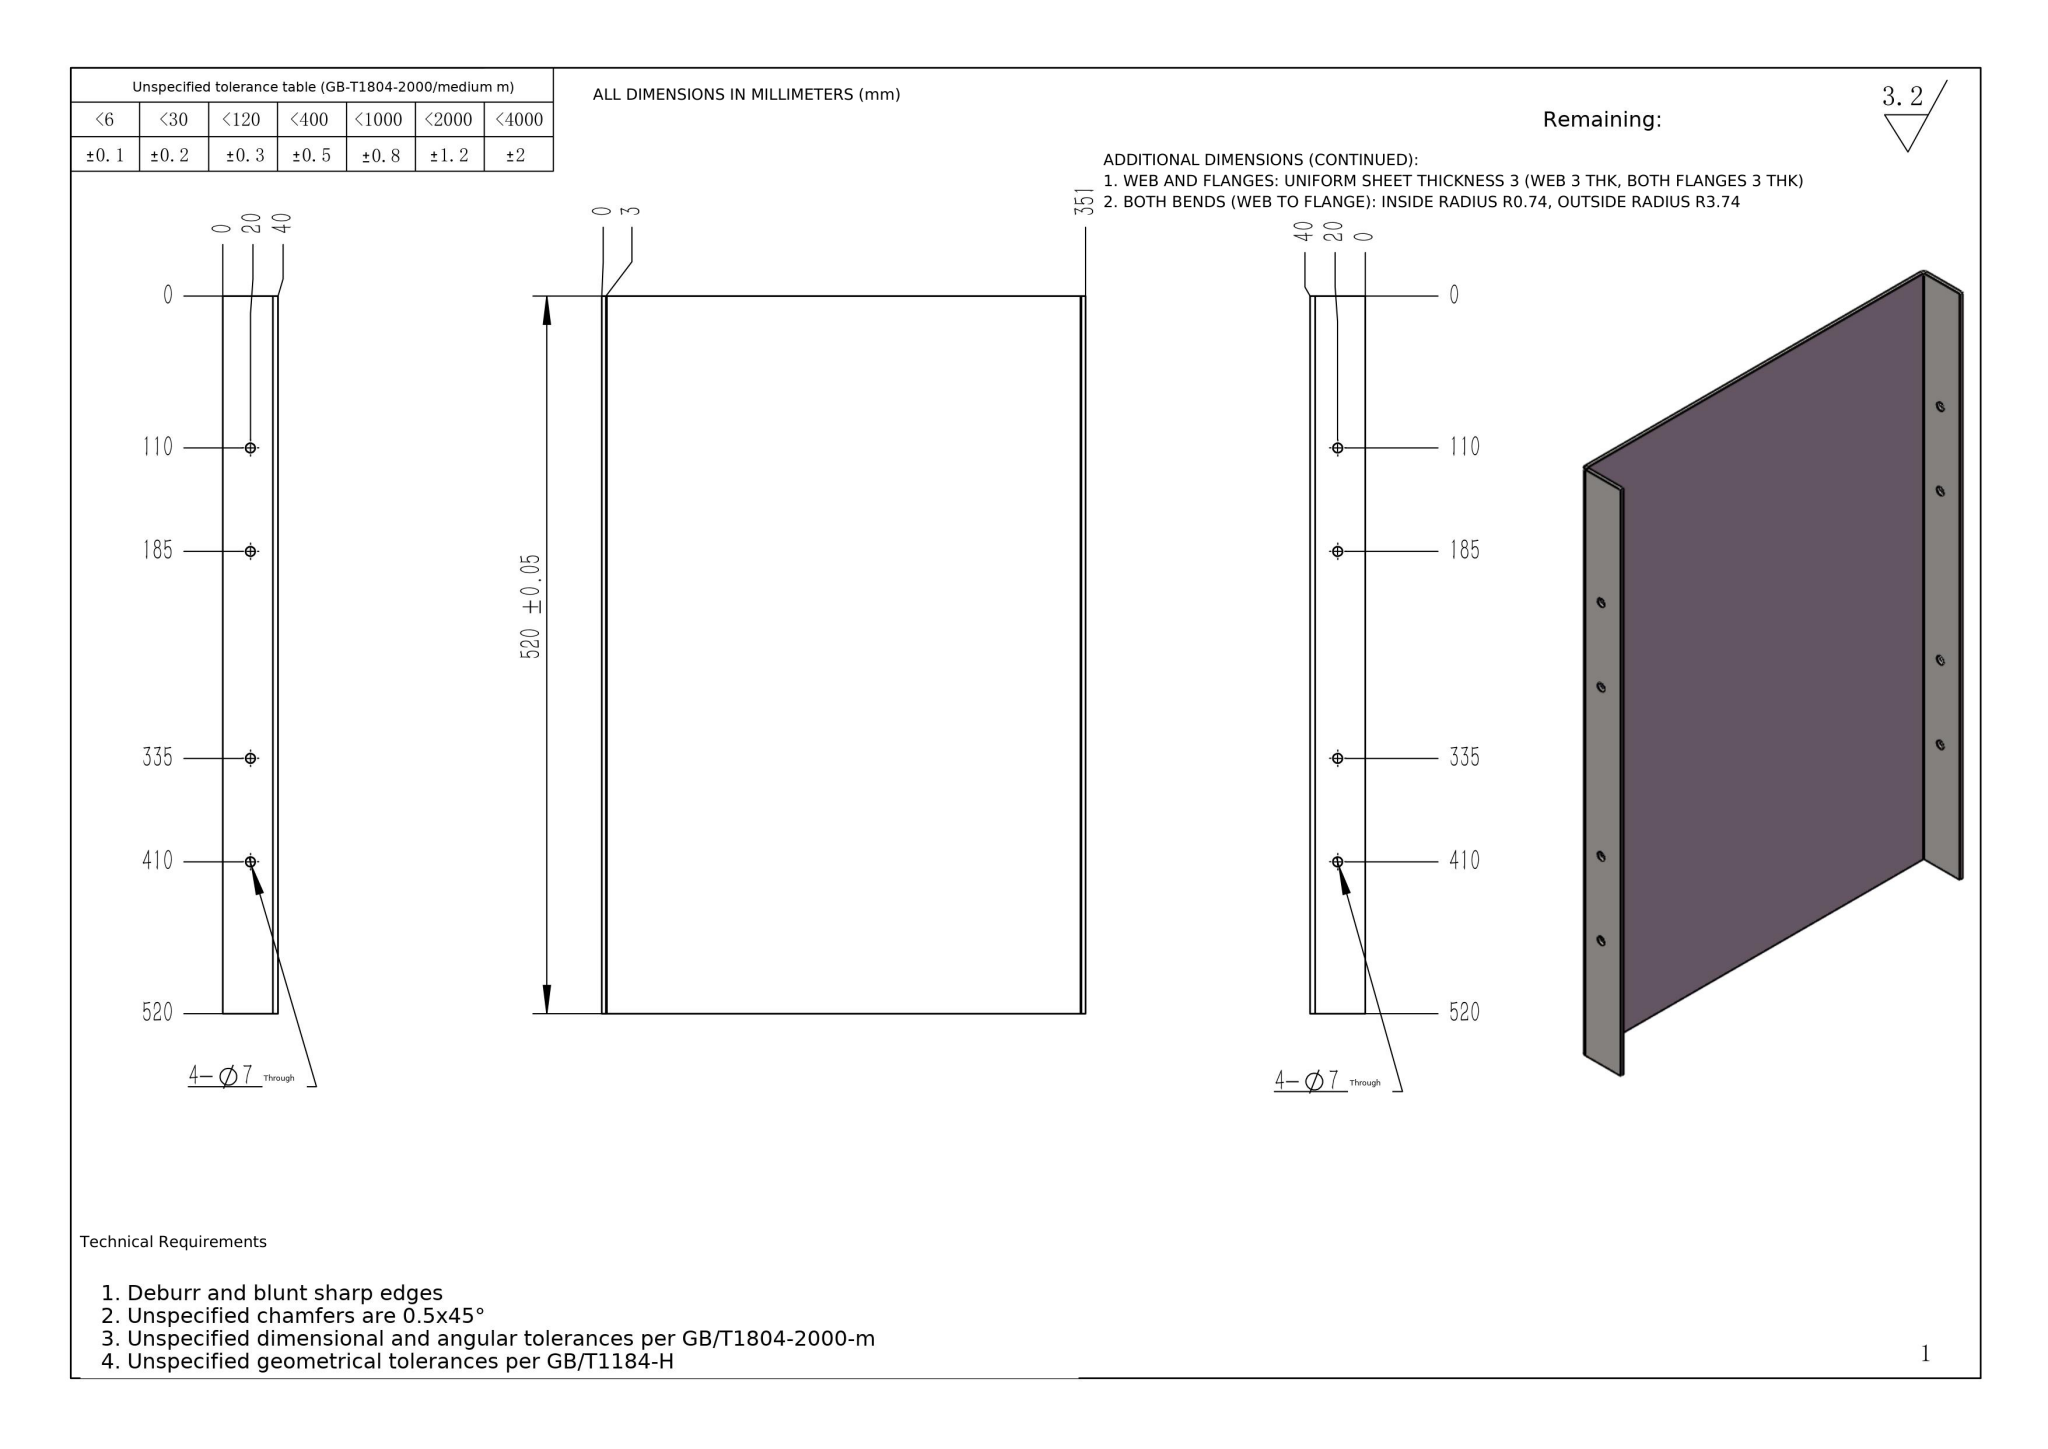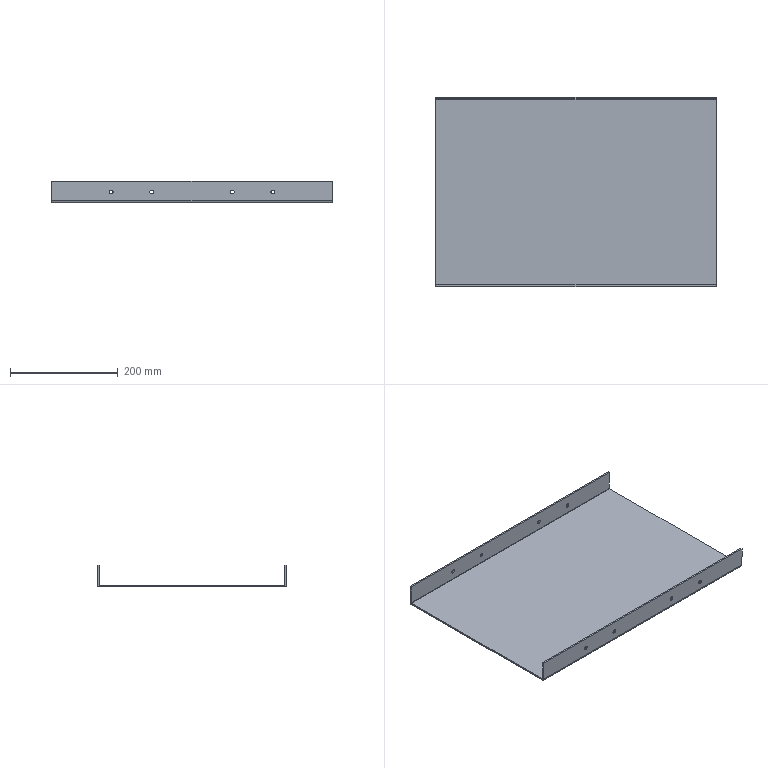Part | NX | mm | 1 solid | 38 faces | box 520 x 351 x 40 mm | volume 659081 mm3 | cylinder 20 | plane 18 | commonest cylinder face diameters 7 x16 7.473 x2 1.473 x2